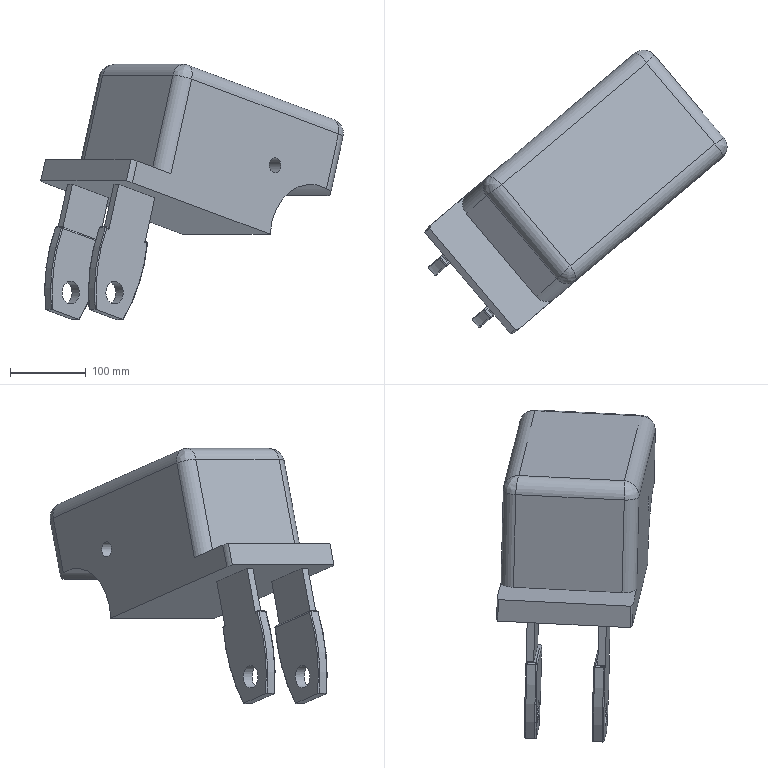Component | NX | BOTA | 1 solid | 78 faces | volume 8839189 mm3 | cylinder 28 | plane 22 | spline 20 | torus 8 | commonest cylinder face diameters 4 x10 40 x6 36 x4 410 x4 30 x2 140 x1 20 x1